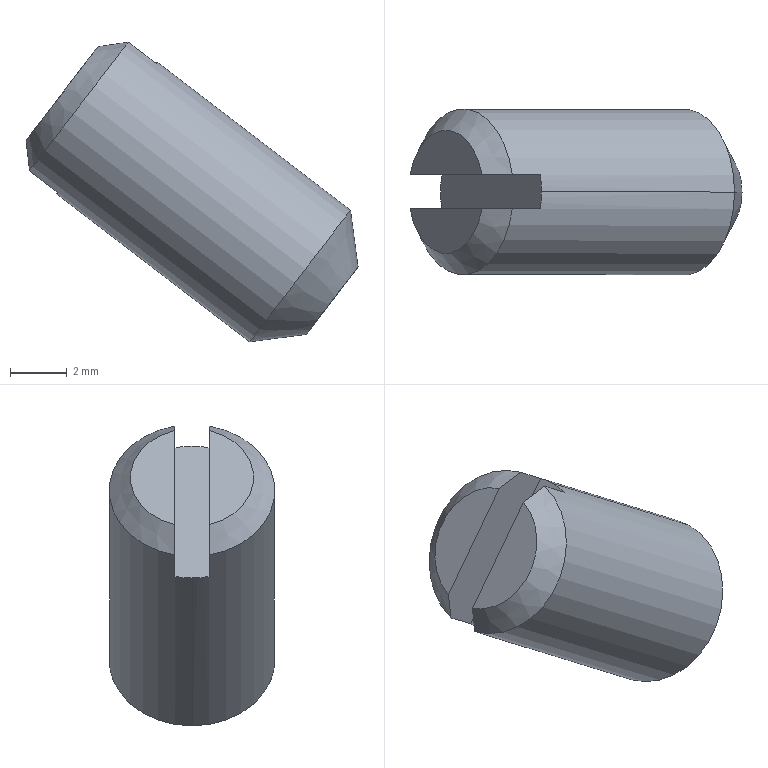Component | SolidWorks | 21-1 | 1 solid | 12 faces | box 11.71 x 5.85 x 10.57 mm | volume 289 mm3 | plane 6 | cone 4 | cylinder 2 | commonest cylinder face diameters 5.847 x2
build123d program:
from build123d import *

# Parameters (mm, degrees)
SKETCH2_W          = 11.616
SKETCH2_H          = 1.2
CUT_EXTRUDE1_DEPTH = 2
CHAMFER1_SIZE      = 0.75


with BuildPart() as part:
    # Sketch1 → Revolve1 (revolve)
    with BuildSketch(Plane(origin=(0, 0, 0), x_dir=(1, 0, 0), z_dir=(0, 1, 0)), mode=Mode.PRIVATE) as revolve1_sk:
        Polygon((0, 0), (0, 2.923), (-10.577, 2.923), (-12, 1.5), (-12, 0), align=None)
    revolve(revolve1_sk.sketch.rotate(Axis((-12, 0, 0), (1, 0, 0)), 180), axis=Axis((-12, 0, 0), (1, 0, 0)))

    # Sketch2 → Cut-Extrude1 (cut)
    with BuildSketch(Plane(origin=(0, 0, 0), x_dir=(0, 0, -1), z_dir=(1, 0, 0))):
        Rectangle(SKETCH2_W, SKETCH2_H)
    extrude(amount=-CUT_EXTRUDE1_DEPTH, mode=Mode.SUBTRACT)

    # Chamfer1
    chamfer1_edges = [part.edges().sort_by_distance(p)[0] for p in [
        (0, -2.923, 0),
        (0, 2.923, 0),
    ]]
    chamfer(chamfer1_edges, length=CHAMFER1_SIZE)


solid = part.part

# Placed as in the assembly
solid = solid.moved(Location((-21.433, -30.7, 16.42), (-180, -37.456, -180)))
STEP:
#1=COLOUR_RGB('',0.7922,0.8196,0.9333);
#2=FILL_AREA_STYLE_COLOUR('',#1);
#3=FILL_AREA_STYLE('',(#2));
#4=SURFACE_STYLE_FILL_AREA(#3);
#5=SURFACE_SIDE_STYLE('',(#4));
#6=SURFACE_STYLE_USAGE(.BOTH.,#5);
#7=PRESENTATION_STYLE_ASSIGNMENT((#6));
#8=CARTESIAN_POINT('',(-0.5047,-1.209,0.3123));
#9=VERTEX_POINT('',#8);
#10=CARTESIAN_POINT('',(-0.4329,-1.209,0.406));
#11=VERTEX_POINT('',#10);
#12=CARTESIAN_POINT('',(-0.4688,-1.209,0.3591));
#13=DIRECTION('',(0.7938,0.,-0.6082));
#14=DIRECTION('',(-0.6082,0.,-0.7938));
#15=AXIS2_PLACEMENT_3D('',#12,#13,#14);
#16=CIRCLE('',#15,0.05906);
#17=EDGE_CURVE('',#9,#11,#16,.T.);
#18=ORIENTED_EDGE('',*,*,#17,.F.);
#19=CARTESIAN_POINT('',(-0.5833,-1.209,0.3019));
#20=VERTEX_POINT('',#19);
#21=CARTESIAN_POINT('',(-0.5833,-1.209,0.3019));
#22=DIRECTION('',(-0.9913,0.,-0.1313));
#23=VECTOR('',#22,39.37);
#24=LINE('',#21,#23);
#25=EDGE_CURVE('',#9,#20,#24,.T.);
#26=ORIENTED_EDGE('',*,*,#25,.T.);
#27=CARTESIAN_POINT('',(-0.4433,-1.209,0.4846));
#28=VERTEX_POINT('',#27);
#29=CARTESIAN_POINT('',(-0.5133,-1.209,0.3932));
#30=DIRECTION('',(0.7938,0.,-0.6082));
#31=DIRECTION('',(-0.6082,0.,-0.7938));
#32=AXIS2_PLACEMENT_3D('',#29,#30,#31);
#33=CIRCLE('',#32,0.1151);
#34=EDGE_CURVE('',#20,#28,#33,.T.);
#35=ORIENTED_EDGE('',*,*,#34,.T.);
#36=CARTESIAN_POINT('',(-0.4433,-1.209,0.4846));
#37=DIRECTION('',(-0.1313,-0.,0.9913));
#38=VECTOR('',#37,39.37);
#39=LINE('',#36,#38);
#40=EDGE_CURVE('',#11,#28,#39,.T.);
#41=ORIENTED_EDGE('',*,*,#40,.F.);
#42=EDGE_LOOP('',(#18,#26,#35,#41));
#43=FACE_OUTER_BOUND('',#42,.T.);
#44=CARTESIAN_POINT('',(-0.5133,-1.209,0.3932));
#45=DIRECTION('',(-0.7938,-0.,0.6082));
#46=DIRECTION('',(0.6082,0.,0.7938));
#47=AXIS2_PLACEMENT_3D('',#44,#45,#46);
#48=CONICAL_SURFACE('',#47,0.1151,0.7854);
#49=ADVANCED_FACE('',(#43),#48,.T.);
#50=CARTESIAN_POINT('',(-0.7128,-1.185,0.688));
#51=VERTEX_POINT('',#50);
#52=CARTESIAN_POINT('',(-0.7113,-1.209,0.6899));
#53=VERTEX_POINT('',#52);
#54=CARTESIAN_POINT('',(-0.7813,-1.209,0.5986));
#55=DIRECTION('',(0.7938,0.,-0.6082));
#56=DIRECTION('',(-0.6082,0.,-0.7938));
#57=AXIS2_PLACEMENT_3D('',#54,#55,#56);
#58=CIRCLE('',#57,0.1151);
#59=EDGE_CURVE('',#51,#53,#58,.T.);
#60=ORIENTED_EDGE('',*,*,#59,.T.);
#61=CARTESIAN_POINT('',(-0.3988,-1.209,0.4505));
#62=DIRECTION('',(0.7938,0.,-0.6082));
#63=VECTOR('',#62,39.37);
#64=LINE('',#61,#63);
#65=EDGE_CURVE('',#53,#28,#64,.T.);
#66=ORIENTED_EDGE('',*,*,#65,.T.);
#67=ORIENTED_EDGE('',*,*,#34,.F.);
#68=CARTESIAN_POINT('',(-0.8513,-1.209,0.5072));
#69=VERTEX_POINT('',#68);
#70=CARTESIAN_POINT('',(-0.5388,-1.209,0.2678));
#71=DIRECTION('',(0.7938,0.,-0.6082));
#72=VECTOR('',#71,39.37);
#73=LINE('',#70,#72);
#74=EDGE_CURVE('',#69,#20,#73,.T.);
#75=ORIENTED_EDGE('',*,*,#74,.F.);
#76=CARTESIAN_POINT('',(-0.8498,-1.185,0.5092));
#77=VERTEX_POINT('',#76);
#78=CARTESIAN_POINT('',(-0.7813,-1.209,0.5986));
#79=DIRECTION('',(0.7938,0.,-0.6082));
#80=DIRECTION('',(-0.6082,0.,-0.7938));
#81=AXIS2_PLACEMENT_3D('',#78,#79,#80);
#82=CIRCLE('',#81,0.1151);
#83=EDGE_CURVE('',#69,#77,#82,.T.);
#84=ORIENTED_EDGE('',*,*,#83,.T.);
#85=CARTESIAN_POINT('',(-0.8889,-1.185,0.5391));
#86=VERTEX_POINT('',#85);
#87=CARTESIAN_POINT('',(-0.5373,-1.185,0.2697));
#88=DIRECTION('',(-0.7938,-0.,0.6082));
#89=VECTOR('',#88,39.37);
#90=LINE('',#87,#89);
#91=EDGE_CURVE('',#77,#86,#90,.T.);
#92=ORIENTED_EDGE('',*,*,#91,.T.);
#93=CARTESIAN_POINT('',(-0.7519,-1.185,0.7179));
#94=VERTEX_POINT('',#93);
#95=CARTESIAN_POINT('',(-0.8204,-1.209,0.6285));
#96=DIRECTION('',(0.7938,0.,-0.6082));
#97=DIRECTION('',(-0.6082,0.,-0.7938));
#98=AXIS2_PLACEMENT_3D('',#95,#96,#97);
#99=CIRCLE('',#98,0.1151);
#100=EDGE_CURVE('',#86,#94,#99,.T.);
#101=ORIENTED_EDGE('',*,*,#100,.T.);
#102=CARTESIAN_POINT('',(-0.4003,-1.185,0.4486));
#103=DIRECTION('',(0.7938,0.,-0.6082));
#104=VECTOR('',#103,39.37);
#105=LINE('',#102,#104);
#106=EDGE_CURVE('',#94,#51,#105,.T.);
#107=ORIENTED_EDGE('',*,*,#106,.T.);
#108=EDGE_LOOP('',(#60,#66,#67,#75,#84,#92,#101,#107));
#109=FACE_OUTER_BOUND('',#108,.T.);
#110=CARTESIAN_POINT('',(-0.4688,-1.209,0.3591));
#111=DIRECTION('',(0.7938,0.,-0.6082));
#112=DIRECTION('',(-0.6082,0.,-0.7938));
#113=AXIS2_PLACEMENT_3D('',#110,#111,#112);
#114=CYLINDRICAL_SURFACE('',#113,0.1151);
#115=ADVANCED_FACE('',(#109),#114,.T.);
#116=CARTESIAN_POINT('',(-0.8938,-1.232,0.5812));
#117=VERTEX_POINT('',#116);
#118=CARTESIAN_POINT('',(-0.7938,-1.232,0.7117));
#119=VERTEX_POINT('',#118);
#120=CARTESIAN_POINT('',(-0.9829,-1.232,0.4649));
#121=DIRECTION('',(0.6082,-0.,0.7938));
#122=VECTOR('',#121,39.37);
#123=LINE('',#120,#122);
#124=EDGE_CURVE('',#117,#119,#123,.T.);
#125=ORIENTED_EDGE('',*,*,#124,.F.);
#126=CARTESIAN_POINT('',(-0.8438,-1.209,0.6465));
#127=DIRECTION('',(-0.7938,-0.,0.6082));
#128=DIRECTION('',(-0.6082,0.,-0.7938));
#129=AXIS2_PLACEMENT_3D('',#126,#127,#128);
#130=CIRCLE('',#129,0.08557);
#131=EDGE_CURVE('',#117,#119,#130,.T.);
#132=ORIENTED_EDGE('',*,*,#131,.T.);
#133=EDGE_LOOP('',(#125,#132));
#134=FACE_OUTER_BOUND('',#133,.T.);
#135=CARTESIAN_POINT('',(-0.8438,-1.209,0.6465));
#136=DIRECTION('',(0.7938,0.,-0.6082));
#137=DIRECTION('',(-0.6082,0.,-0.7938));
#138=AXIS2_PLACEMENT_3D('',#135,#136,#137);
#139=PLANE('',#138);
#140=ADVANCED_FACE('',(#134),#139,.F.);
#141=CARTESIAN_POINT('',(-0.7938,-1.185,0.7117));
#142=VERTEX_POINT('',#141);
#143=CARTESIAN_POINT('',(-0.8938,-1.185,0.5812));
#144=VERTEX_POINT('',#143);
#145=CARTESIAN_POINT('',(-0.9829,-1.185,0.4649));
#146=DIRECTION('',(-0.6082,0.,-0.7938));
#147=VECTOR('',#146,39.37);
#148=LINE('',#145,#147);
#149=EDGE_CURVE('',#142,#144,#148,.T.);
#150=ORIENTED_EDGE('',*,*,#149,.F.);
#151=CARTESIAN_POINT('',(-0.8438,-1.209,0.6465));
#152=DIRECTION('',(-0.7938,-0.,0.6082));
#153=DIRECTION('',(-0.6082,0.,-0.7938));
#154=AXIS2_PLACEMENT_3D('',#151,#152,#153);
#155=CIRCLE('',#154,0.08557);
#156=EDGE_CURVE('',#142,#144,#155,.T.);
#157=ORIENTED_EDGE('',*,*,#156,.T.);
#158=EDGE_LOOP('',(#150,#157));
#159=FACE_OUTER_BOUND('',#158,.T.);
#160=CARTESIAN_POINT('',(-0.8438,-1.209,0.6465));
#161=DIRECTION('',(0.7938,0.,-0.6082));
#162=DIRECTION('',(-0.6082,0.,-0.7938));
#163=AXIS2_PLACEMENT_3D('',#160,#161,#162);
#164=PLANE('',#163);
#165=ADVANCED_FACE('',(#159),#164,.F.);
#166=ORIENTED_EDGE('',*,*,#65,.F.);
#167=CARTESIAN_POINT('',(-0.7128,-1.232,0.688));
#168=VERTEX_POINT('',#167);
#169=CARTESIAN_POINT('',(-0.7813,-1.209,0.5986));
#170=DIRECTION('',(0.7938,0.,-0.6082));
#171=DIRECTION('',(-0.6082,0.,-0.7938));
#172=AXIS2_PLACEMENT_3D('',#169,#170,#171);
#173=CIRCLE('',#172,0.1151);
#174=EDGE_CURVE('',#53,#168,#173,.T.);
#175=ORIENTED_EDGE('',*,*,#174,.T.);
#176=CARTESIAN_POINT('',(-0.7519,-1.232,0.7179));
#177=VERTEX_POINT('',#176);
#178=CARTESIAN_POINT('',(-0.4003,-1.232,0.4486));
#179=DIRECTION('',(-0.7938,-0.,0.6082));
#180=VECTOR('',#179,39.37);
#181=LINE('',#178,#180);
#182=EDGE_CURVE('',#168,#177,#181,.T.);
#183=ORIENTED_EDGE('',*,*,#182,.T.);
#184=CARTESIAN_POINT('',(-0.8889,-1.232,0.5391));
#185=VERTEX_POINT('',#184);
#186=CARTESIAN_POINT('',(-0.8204,-1.209,0.6285));
#187=DIRECTION('',(0.7938,0.,-0.6082));
#188=DIRECTION('',(-0.6082,0.,-0.7938));
#189=AXIS2_PLACEMENT_3D('',#186,#187,#188);
#190=CIRCLE('',#189,0.1151);
#191=EDGE_CURVE('',#177,#185,#190,.T.);
#192=ORIENTED_EDGE('',*,*,#191,.T.);
#193=CARTESIAN_POINT('',(-0.8498,-1.232,0.5092));
#194=VERTEX_POINT('',#193);
#195=CARTESIAN_POINT('',(-0.5373,-1.232,0.2697));
#196=DIRECTION('',(0.7938,0.,-0.6082));
#197=VECTOR('',#196,39.37);
#198=LINE('',#195,#197);
#199=EDGE_CURVE('',#185,#194,#198,.T.);
#200=ORIENTED_EDGE('',*,*,#199,.T.);
#201=CARTESIAN_POINT('',(-0.7813,-1.209,0.5986));
#202=DIRECTION('',(0.7938,0.,-0.6082));
#203=DIRECTION('',(-0.6082,0.,-0.7938));
#204=AXIS2_PLACEMENT_3D('',#201,#202,#203);
#205=CIRCLE('',#204,0.1151);
#206=EDGE_CURVE('',#194,#69,#205,.T.);
#207=ORIENTED_EDGE('',*,*,#206,.T.);
#208=ORIENTED_EDGE('',*,*,#74,.T.);
#209=CARTESIAN_POINT('',(-0.5133,-1.209,0.3932));
#210=DIRECTION('',(0.7938,0.,-0.6082));
#211=DIRECTION('',(-0.6082,0.,-0.7938));
#212=AXIS2_PLACEMENT_3D('',#209,#210,#211);
#213=CIRCLE('',#212,0.1151);
#214=EDGE_CURVE('',#28,#20,#213,.T.);
#215=ORIENTED_EDGE('',*,*,#214,.F.);
#216=EDGE_LOOP('',(#166,#175,#183,#192,#200,#207,#208,#215));
#217=FACE_OUTER_BOUND('',#216,.T.);
#218=CARTESIAN_POINT('',(-0.4688,-1.209,0.3591));
#219=DIRECTION('',(0.7938,0.,-0.6082));
#220=DIRECTION('',(-0.6082,0.,-0.7938));
#221=AXIS2_PLACEMENT_3D('',#218,#219,#220);
#222=CYLINDRICAL_SURFACE('',#221,0.1151);
#223=ADVANCED_FACE('',(#217),#222,.T.);
#224=ORIENTED_EDGE('',*,*,#25,.F.);
#225=CARTESIAN_POINT('',(-0.4688,-1.209,0.3591));
#226=DIRECTION('',(0.7938,0.,-0.6082));
#227=DIRECTION('',(-0.6082,0.,-0.7938));
#228=AXIS2_PLACEMENT_3D('',#225,#226,#227);
#229=CIRCLE('',#228,0.05906);
#230=EDGE_CURVE('',#11,#9,#229,.T.);
#231=ORIENTED_EDGE('',*,*,#230,.F.);
#232=ORIENTED_EDGE('',*,*,#40,.T.);
#233=ORIENTED_EDGE('',*,*,#214,.T.);
#234=EDGE_LOOP('',(#224,#231,#232,#233));
#235=FACE_OUTER_BOUND('',#234,.T.);
#236=CARTESIAN_POINT('',(-0.5133,-1.209,0.3932));
#237=DIRECTION('',(-0.7938,-0.,0.6082));
#238=DIRECTION('',(0.6082,0.,0.7938));
#239=AXIS2_PLACEMENT_3D('',#236,#237,#238);
#240=CONICAL_SURFACE('',#239,0.1151,0.7854);
#241=ADVANCED_FACE('',(#235),#240,.T.);
#242=ORIENTED_EDGE('',*,*,#230,.T.);
#243=ORIENTED_EDGE('',*,*,#17,.T.);
#244=EDGE_LOOP('',(#242,#243));
#245=FACE_OUTER_BOUND('',#244,.T.);
#246=CARTESIAN_POINT('',(-0.4329,-1.209,0.406));
#247=DIRECTION('',(-0.7938,-0.,0.6082));
#248=DIRECTION('',(0.6082,-0.,0.7938));
#249=AXIS2_PLACEMENT_3D('',#246,#247,#248);
#250=PLANE('',#249);
#251=ADVANCED_FACE('',(#245),#250,.F.);
#252=ORIENTED_EDGE('',*,*,#199,.F.);
#253=CARTESIAN_POINT('',(-0.8889,-1.232,0.5391));
#254=CARTESIAN_POINT('',(-0.8906,-1.232,0.5531));
#255=CARTESIAN_POINT('',(-0.8923,-1.232,0.5671));
#256=CARTESIAN_POINT('',(-0.8938,-1.232,0.5812));
#257=B_SPLINE_CURVE_WITH_KNOTS('',3,(#253,#254,#255,#256),.UNSPECIFIED.,.F.,.F.,(4,4),(0.,0.001076),.UNSPECIFIED.);
#258=EDGE_CURVE('',#185,#117,#257,.T.);
#259=ORIENTED_EDGE('',*,*,#258,.T.);
#260=ORIENTED_EDGE('',*,*,#124,.T.);
#261=CARTESIAN_POINT('',(-0.7938,-1.232,0.7117));
#262=CARTESIAN_POINT('',(-0.7798,-1.232,0.7139));
#263=CARTESIAN_POINT('',(-0.7659,-1.232,0.7159));
#264=CARTESIAN_POINT('',(-0.7519,-1.232,0.7179));
#265=B_SPLINE_CURVE_WITH_KNOTS('',3,(#261,#262,#263,#264),.UNSPECIFIED.,.F.,.F.,(4,4),(0.,0.001076),.UNSPECIFIED.);
#266=EDGE_CURVE('',#119,#177,#265,.T.);
#267=ORIENTED_EDGE('',*,*,#266,.T.);
#268=ORIENTED_EDGE('',*,*,#182,.F.);
#269=CARTESIAN_POINT('',(-0.9204,-1.232,0.4171));
#270=DIRECTION('',(0.6082,-0.,0.7938));
#271=VECTOR('',#270,39.37);
#272=LINE('',#269,#271);
#273=EDGE_CURVE('',#194,#168,#272,.T.);
#274=ORIENTED_EDGE('',*,*,#273,.F.);
#275=EDGE_LOOP('',(#252,#259,#260,#267,#268,#274));
#276=FACE_OUTER_BOUND('',#275,.T.);
#277=CARTESIAN_POINT('',(-0.9204,-1.232,0.4171));
#278=DIRECTION('',(0.,-1.,-0.));
#279=DIRECTION('',(0.6082,-0.,0.7938));
#280=AXIS2_PLACEMENT_3D('',#277,#278,#279);
#281=PLANE('',#280);
#282=ADVANCED_FACE('',(#276),#281,.F.);
#283=ORIENTED_EDGE('',*,*,#106,.F.);
#284=CARTESIAN_POINT('',(-0.7519,-1.185,0.7179));
#285=CARTESIAN_POINT('',(-0.7659,-1.185,0.7159));
#286=CARTESIAN_POINT('',(-0.7798,-1.185,0.7139));
#287=CARTESIAN_POINT('',(-0.7938,-1.185,0.7117));
#288=B_SPLINE_CURVE_WITH_KNOTS('',3,(#284,#285,#286,#287),.UNSPECIFIED.,.F.,.F.,(4,4),(0.,0.001076),.UNSPECIFIED.);
#289=EDGE_CURVE('',#94,#142,#288,.T.);
#290=ORIENTED_EDGE('',*,*,#289,.T.);
#291=ORIENTED_EDGE('',*,*,#149,.T.);
#292=CARTESIAN_POINT('',(-0.8938,-1.185,0.5812));
#293=CARTESIAN_POINT('',(-0.8923,-1.185,0.5671));
#294=CARTESIAN_POINT('',(-0.8906,-1.185,0.5531));
#295=CARTESIAN_POINT('',(-0.8889,-1.185,0.5391));
#296=B_SPLINE_CURVE_WITH_KNOTS('',3,(#292,#293,#294,#295),.UNSPECIFIED.,.F.,.F.,(4,4),(0.,0.001076),.UNSPECIFIED.);
#297=EDGE_CURVE('',#144,#86,#296,.T.);
#298=ORIENTED_EDGE('',*,*,#297,.T.);
#299=ORIENTED_EDGE('',*,*,#91,.F.);
#300=CARTESIAN_POINT('',(-0.9204,-1.185,0.4171));
#301=DIRECTION('',(-0.6082,0.,-0.7938));
#302=VECTOR('',#301,39.37);
#303=LINE('',#300,#302);
#304=EDGE_CURVE('',#51,#77,#303,.T.);
#305=ORIENTED_EDGE('',*,*,#304,.F.);
#306=EDGE_LOOP('',(#283,#290,#291,#298,#299,#305));
#307=FACE_OUTER_BOUND('',#306,.T.);
#308=CARTESIAN_POINT('',(-0.9204,-1.185,0.4171));
#309=DIRECTION('',(-0.,1.,0.));
#310=DIRECTION('',(-0.6082,0.,-0.7938));
#311=AXIS2_PLACEMENT_3D('',#308,#309,#310);
#312=PLANE('',#311);
#313=ADVANCED_FACE('',(#307),#312,.F.);
#314=ORIENTED_EDGE('',*,*,#304,.T.);
#315=ORIENTED_EDGE('',*,*,#83,.F.);
#316=ORIENTED_EDGE('',*,*,#206,.F.);
#317=ORIENTED_EDGE('',*,*,#273,.T.);
#318=ORIENTED_EDGE('',*,*,#174,.F.);
#319=ORIENTED_EDGE('',*,*,#59,.F.);
#320=EDGE_LOOP('',(#314,#315,#316,#317,#318,#319));
#321=FACE_OUTER_BOUND('',#320,.T.);
#322=CARTESIAN_POINT('',(-0.7813,-1.209,0.5986));
#323=DIRECTION('',(0.7938,0.,-0.6082));
#324=DIRECTION('',(-0.6082,0.,-0.7938));
#325=AXIS2_PLACEMENT_3D('',#322,#323,#324);
#326=PLANE('',#325);
#327=ADVANCED_FACE('',(#321),#326,.F.);
#328=ORIENTED_EDGE('',*,*,#266,.F.);
#329=ORIENTED_EDGE('',*,*,#131,.F.);
#330=ORIENTED_EDGE('',*,*,#258,.F.);
#331=ORIENTED_EDGE('',*,*,#191,.F.);
#332=EDGE_LOOP('',(#328,#329,#330,#331));
#333=FACE_OUTER_BOUND('',#332,.T.);
#334=CARTESIAN_POINT('',(-0.8204,-1.209,0.6285));
#335=DIRECTION('',(0.7938,0.,-0.6082));
#336=DIRECTION('',(-0.6082,0.,-0.7938));
#337=AXIS2_PLACEMENT_3D('',#334,#335,#336);
#338=CONICAL_SURFACE('',#337,0.1151,0.7854);
#339=ADVANCED_FACE('',(#333),#338,.T.);
#340=ORIENTED_EDGE('',*,*,#297,.F.);
#341=ORIENTED_EDGE('',*,*,#156,.F.);
#342=ORIENTED_EDGE('',*,*,#289,.F.);
#343=ORIENTED_EDGE('',*,*,#100,.F.);
#344=EDGE_LOOP('',(#340,#341,#342,#343));
#345=FACE_OUTER_BOUND('',#344,.T.);
#346=CARTESIAN_POINT('',(-0.8204,-1.209,0.6285));
#347=DIRECTION('',(0.7938,0.,-0.6082));
#348=DIRECTION('',(-0.6082,0.,-0.7938));
#349=AXIS2_PLACEMENT_3D('',#346,#347,#348);
#350=CONICAL_SURFACE('',#349,0.1151,0.7854);
#351=ADVANCED_FACE('',(#345),#350,.T.);
#352=CLOSED_SHELL('',(#49,#115,#140,#165,#223,#241,#251,#282,#313,#327,#339,#351));
#353=MANIFOLD_SOLID_BREP('',#352);
#354=STYLED_ITEM('',(#7),#353);
#355=PRESENTATION_LAYER_ASSIGNMENT('','',(#354));
#356=CARTESIAN_POINT('',(0.,0.,0.));
#357=DIRECTION('',(0.,0.,1.));
#358=DIRECTION('',(1.,0.,0.));
#359=AXIS2_PLACEMENT_3D('',#356,#357,#358);
#360=(LENGTH_UNIT()NAMED_UNIT(*)SI_UNIT($,.METRE.));
#361=LENGTH_MEASURE_WITH_UNIT(LENGTH_MEASURE(0.0254),#360);
#362=DIMENSIONAL_EXPONENTS(1.,0.,0.,0.,0.,0.,0.);
#363=(CONVERSION_BASED_UNIT('',#361)LENGTH_UNIT()NAMED_UNIT(#362));
#364=UNCERTAINTY_MEASURE_WITH_UNIT(LENGTH_MEASURE(0.00001),#363,'','');
#365=(NAMED_UNIT(*)PLANE_ANGLE_UNIT()SI_UNIT($,.RADIAN.));
#366=(NAMED_UNIT(*)SI_UNIT($,.STERADIAN.)SOLID_ANGLE_UNIT());
#367=(GEOMETRIC_REPRESENTATION_CONTEXT(3)GLOBAL_UNCERTAINTY_ASSIGNED_CONTEXT((#364))GLOBAL_UNIT_ASSIGNED_CONTEXT((#363,#365,#366))REPRESENTATION_CONTEXT('',''));
#368=ADVANCED_BREP_SHAPE_REPRESENTATION('',(#353,#359),#367);
#369=(LENGTH_UNIT()NAMED_UNIT(*)SI_UNIT($,.METRE.));
#370=LENGTH_MEASURE_WITH_UNIT(LENGTH_MEASURE(0.0254),#369);
#371=DIMENSIONAL_EXPONENTS(1.,0.,0.,0.,0.,0.,0.);
#372=(CONVERSION_BASED_UNIT('',#370)LENGTH_UNIT()NAMED_UNIT(#371));
#373=UNCERTAINTY_MEASURE_WITH_UNIT(LENGTH_MEASURE(0.00001),#372,'','');
#374=(NAMED_UNIT(*)PLANE_ANGLE_UNIT()SI_UNIT($,.RADIAN.));
#375=(NAMED_UNIT(*)SI_UNIT($,.STERADIAN.)SOLID_ANGLE_UNIT());
#376=(GEOMETRIC_REPRESENTATION_CONTEXT(3)GLOBAL_UNCERTAINTY_ASSIGNED_CONTEXT((#373))GLOBAL_UNIT_ASSIGNED_CONTEXT((#372,#374,#375))REPRESENTATION_CONTEXT('',''));
#377=MECHANICAL_DESIGN_GEOMETRIC_PRESENTATION_REPRESENTATION('',(#354),#376);